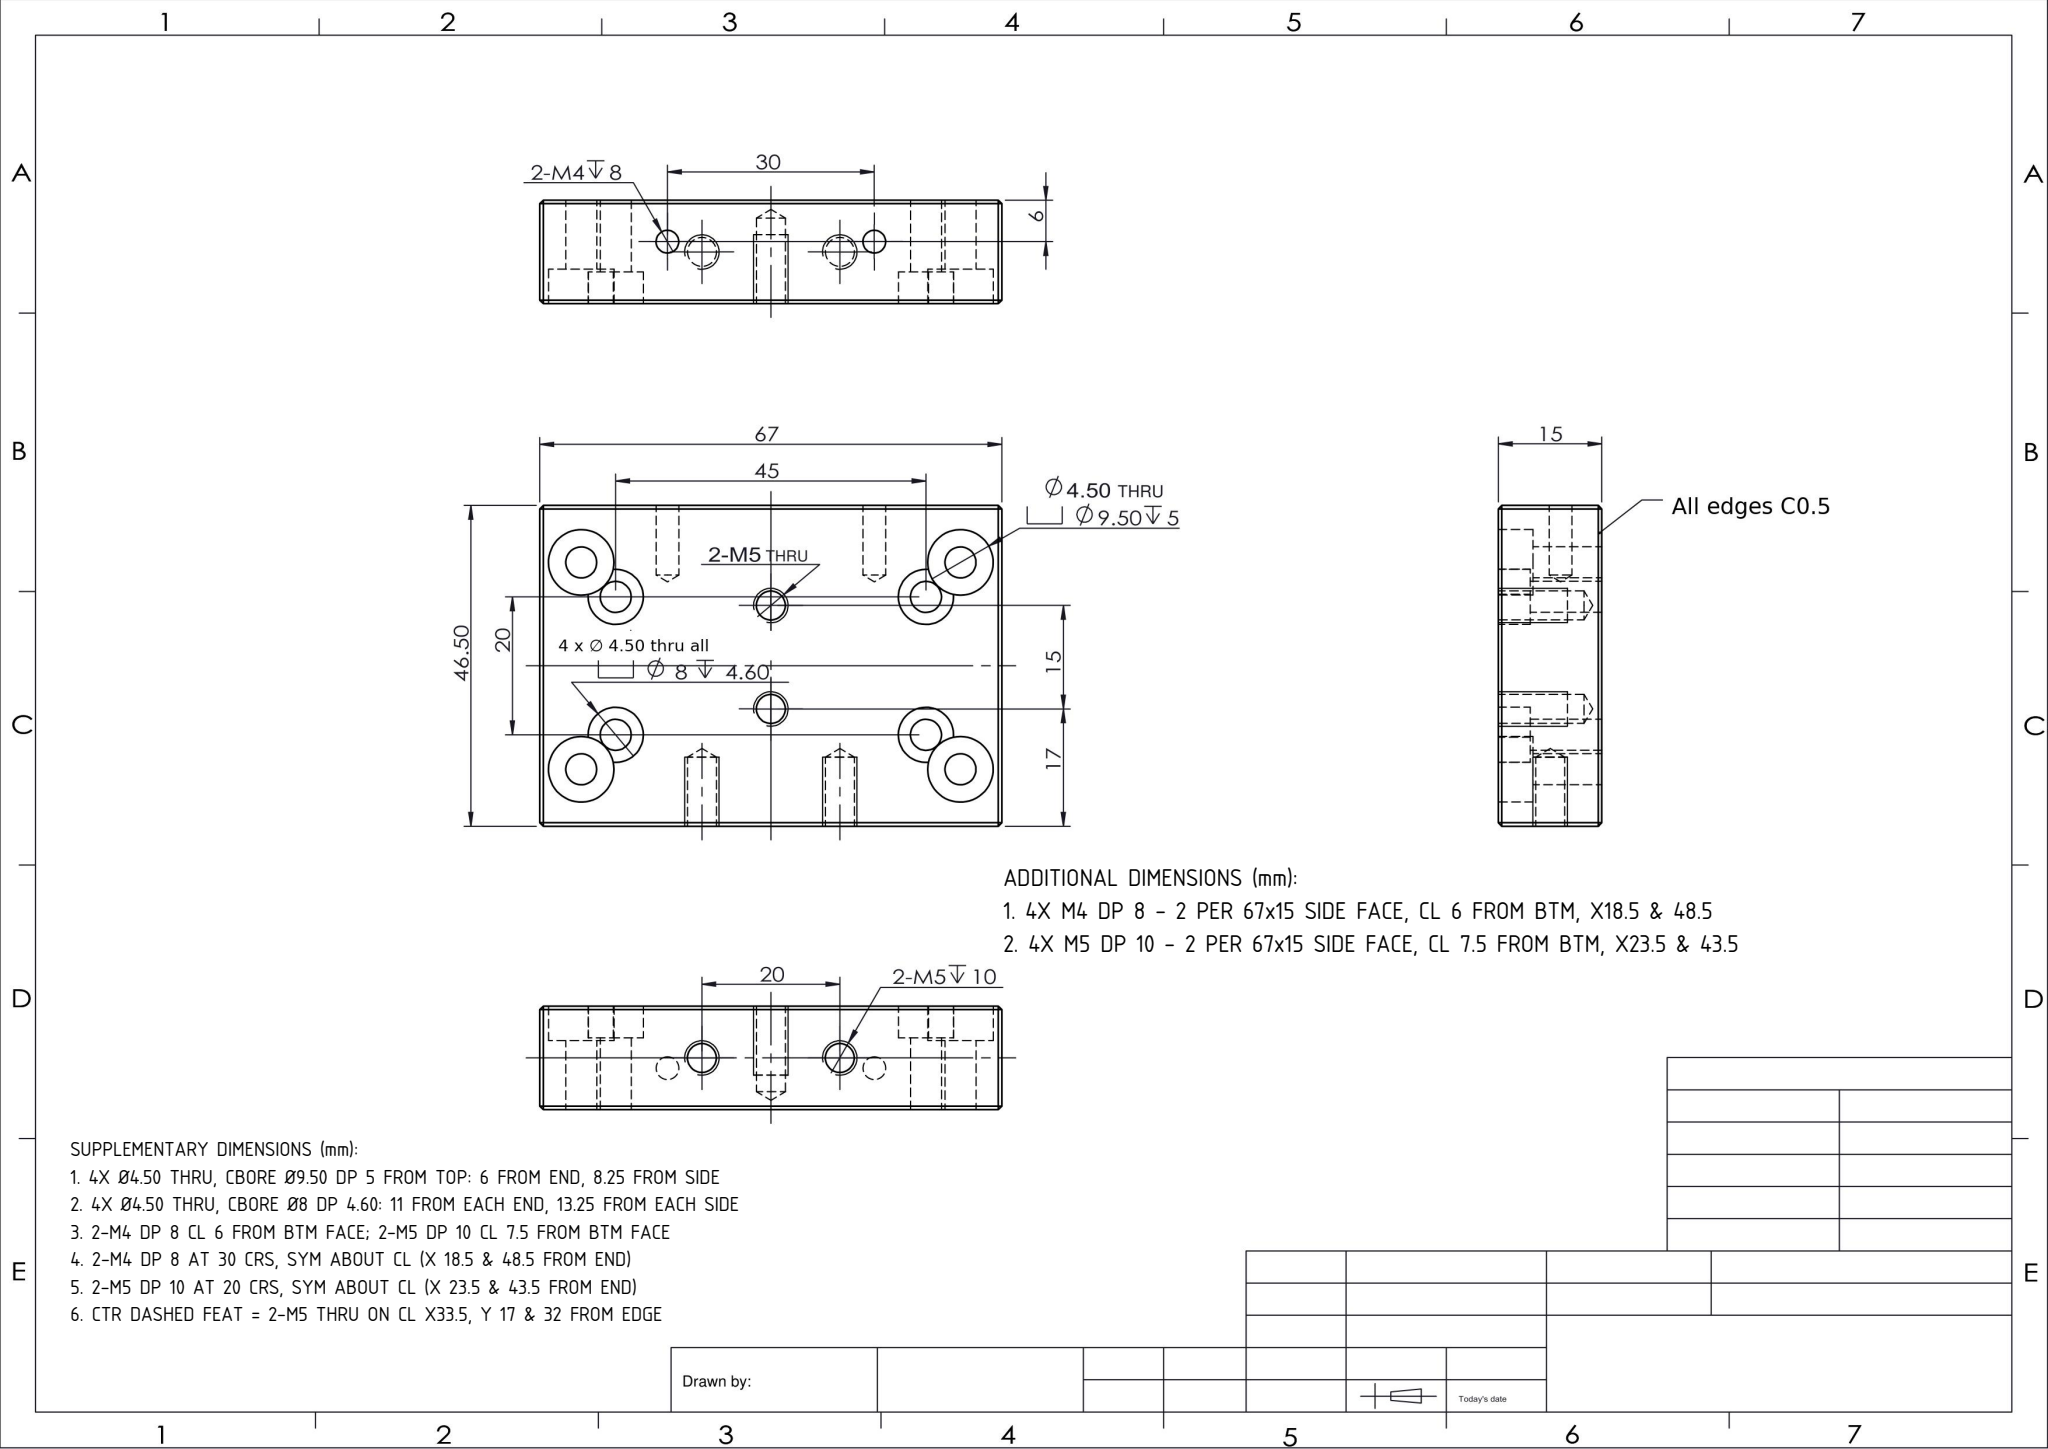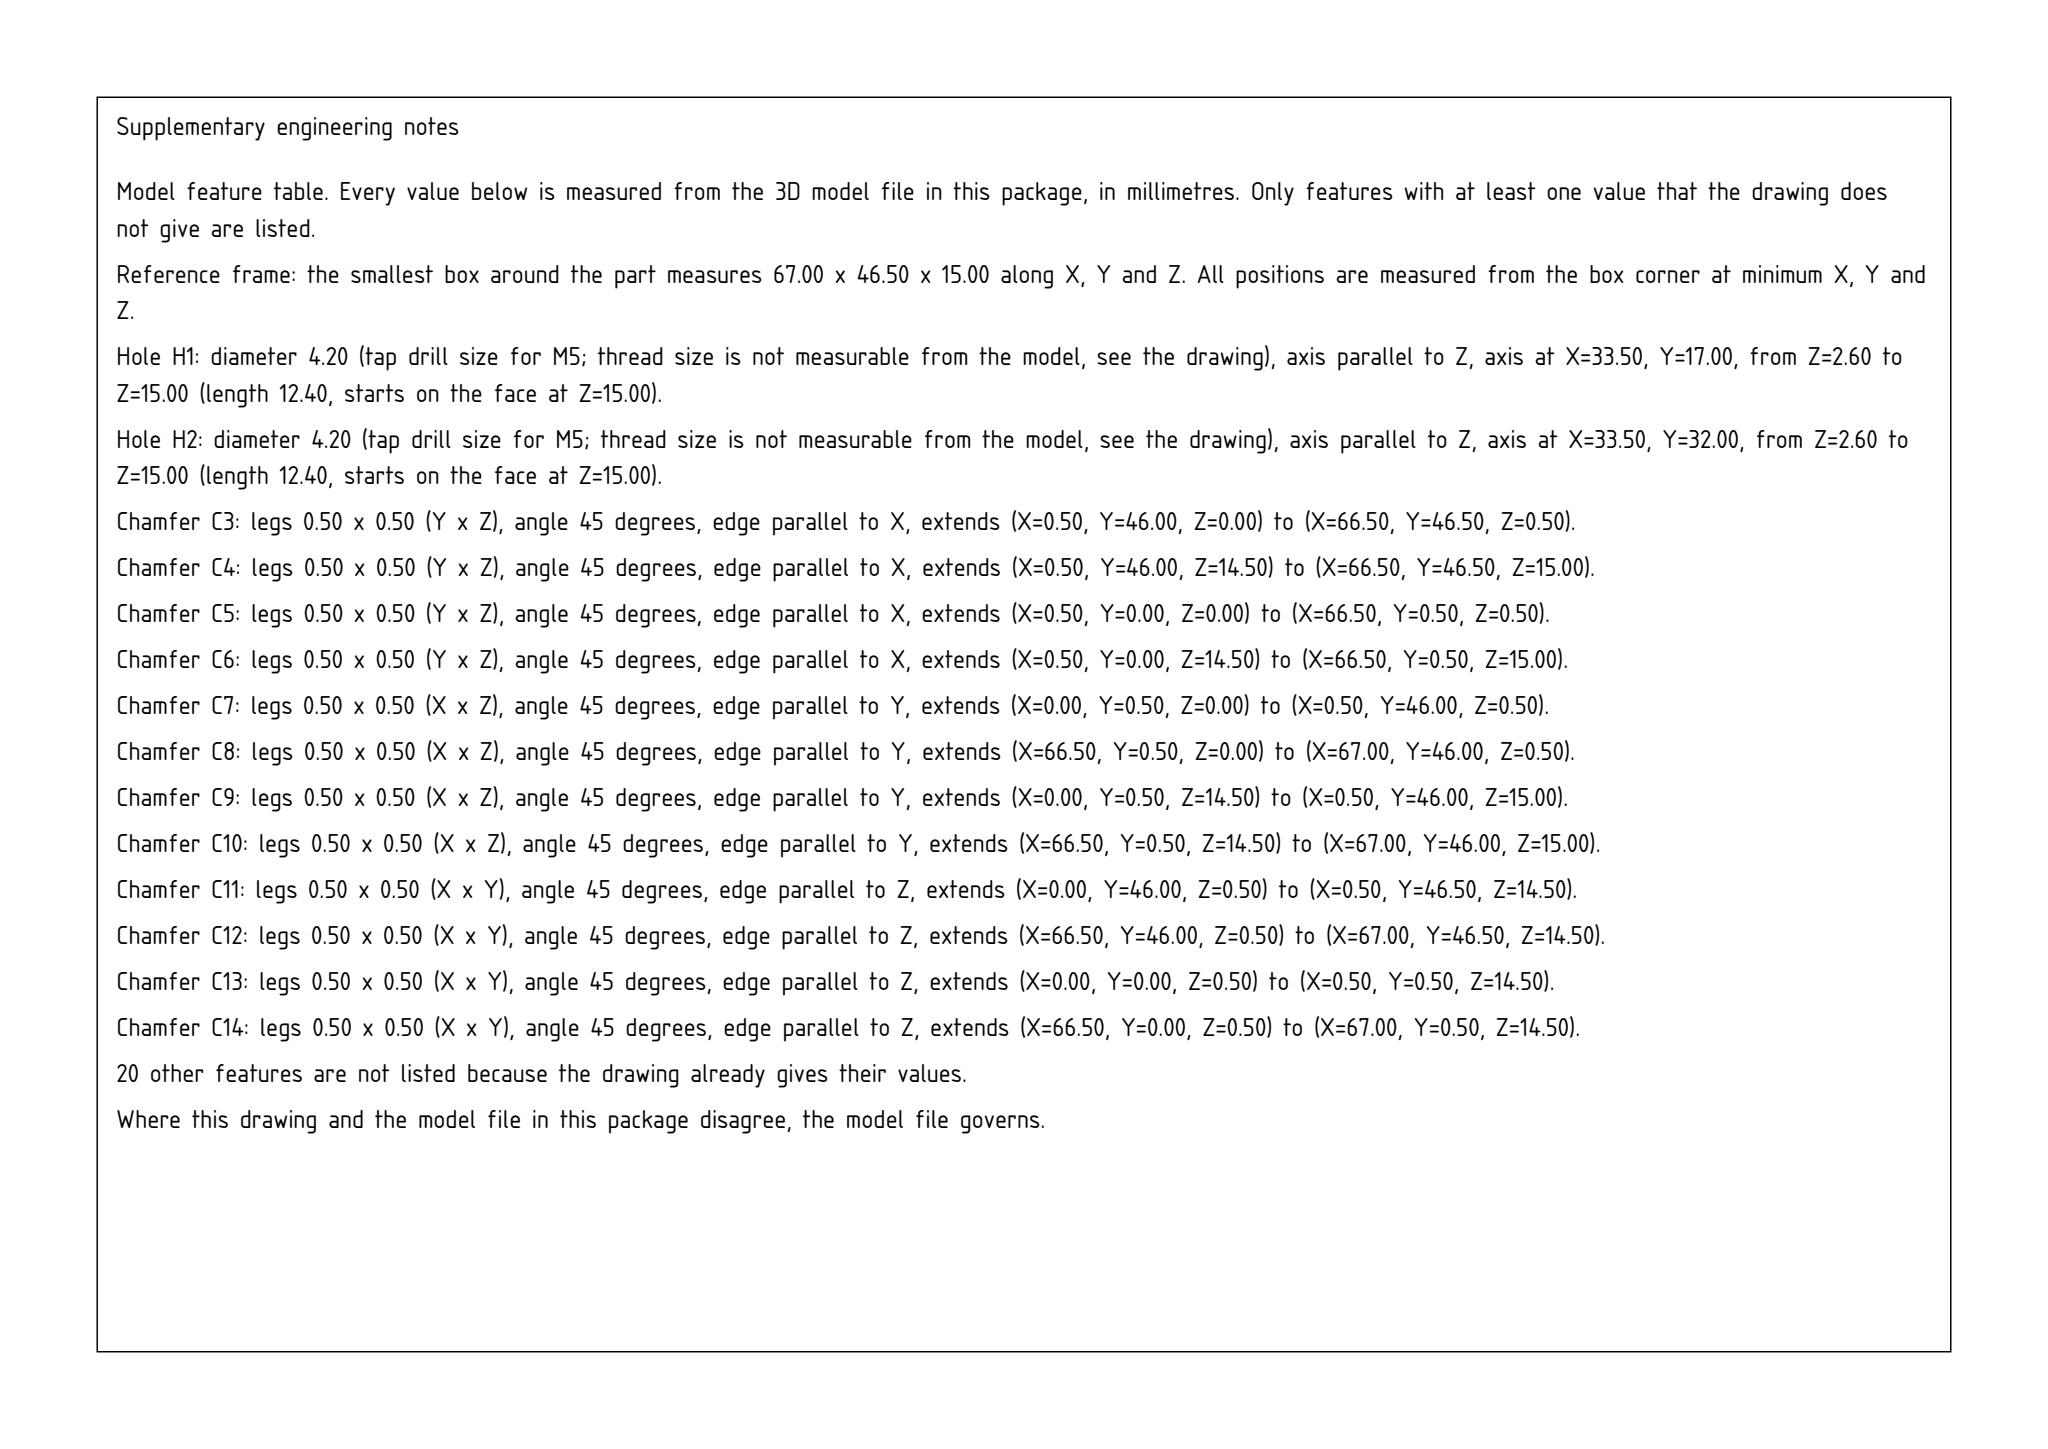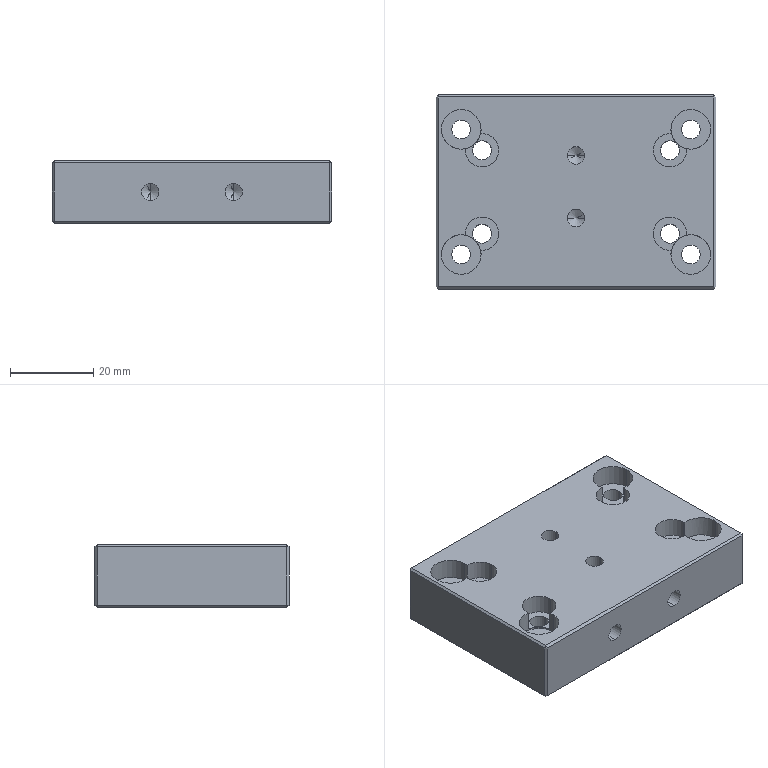Part | SolidWorks | mm | 1 solid | 94 faces | box 67 x 46.5 x 15 mm | volume 42314 mm3 | cylinder 48 | plane 34 | cone 12 | commonest cylinder face diameters 4.5 x16 8 x12 4.2 x8 9.5 x8 3.3 x4
build123d program:
from build123d import *

# Parameters (mm, degrees)
SKETCH1_W                                            = 67
SKETCH1_H                                            = 46.5
BOSS_EXTRUDE1_DEPTH                                  = 7.5
SKETCH2_R                                            = 2.25
CUT_EXTRUDE1_DEPTH                                   = 44.449
SKETCH3_R                                            = 4.75
CUT_EXTRUDE2_DEPTH                                   = 5
CHAMFER1_SIZE                                        = 0.5
M5_TAPPED_HOLE1_D                                    = 4.2
M5_TAPPED_HOLE1_DEPTH                                = 12.4
M5_TAPPED_HOLE1_TIP                                  = 1.262
M5_TAPPED_HOLE2_D                                    = 4.2
M5_TAPPED_HOLE2_DEPTH                                = 10
M5_TAPPED_HOLE2_TIP                                  = 1.262
M4_TAPPED_HOLE1_D                                    = 3.3
M4_TAPPED_HOLE1_DEPTH                                = 10.1
M4_TAPPED_HOLE1_TIP                                  = 0.9914
HOLE_SIZE_ACCORDING_TO_HEXAGON_SOCKET_HE_D           = 4.5
HOLE_SIZE_ACCORDING_TO_HEXAGON_SOCKET_HE_CBORE_D     = 8
HOLE_SIZE_ACCORDING_TO_HEXAGON_SOCKET_HE_CBORE_DEPTH = 4.6


with BuildPart() as part:
    # Sketch1 → Boss-Extrude1 (new, symmetric)
    with BuildSketch(Plane.XY):
        Rectangle(SKETCH1_W, SKETCH1_H)
    extrude(amount=BOSS_EXTRUDE1_DEPTH, both=True)

    # Sketch2 → Cut-Extrude1 (cut, through all)
    with BuildSketch(Plane.XY.offset(7.5)):
        with Locations((-27.5, 15)):
            Circle(SKETCH2_R)
        with Locations(Location((27.5, 15, 0), (0, 0, 180))):
            Circle(SKETCH2_R)
        with Locations((27.5, -15)):
            Circle(SKETCH2_R)
        with Locations(Location((-27.5, -15, 0), (0, 0, 180))):
            Circle(SKETCH2_R)
    extrude(amount=-CUT_EXTRUDE1_DEPTH, mode=Mode.SUBTRACT)

    # Sketch3 → Cut-Extrude2 (cut)
    with BuildSketch(Plane.XY.offset(7.5)):
        with Locations((-27.5, 15)):
            Circle(SKETCH3_R)
        with Locations((27.5, 15)):
            Circle(SKETCH3_R)
        with Locations((-27.5, -15)):
            Circle(SKETCH3_R)
        with Locations((27.5, -15)):
            Circle(SKETCH3_R)
    extrude(amount=-CUT_EXTRUDE2_DEPTH, mode=Mode.SUBTRACT)

    # Chamfer1
    chamfer1_edges = [part.edges().sort_by_distance(p)[0] for p in [
        (-33.5, 0, 7.5),
        (0, -23.25, 7.5),
        (33.5, 0, 7.5),
        (0, -23.25, -7.5),
        (-33.5, 0, -7.5),
        (0, 23.25, -7.5),
        (33.5, 0, -7.5),
        (0, 23.25, 7.5),
        (33.5, -23.25, 0),
        (-33.5, -23.25, 0),
        (-33.5, 23.25, 0),
        (33.5, 23.25, 0),
    ]]
    chamfer(chamfer1_edges, length=CHAMFER1_SIZE)

    # M5 Tapped Hole1
    with Locations(Plane.XY.offset(7.5)):
        with Locations((0, -6.25), (0, 8.75)):
            Hole(M5_TAPPED_HOLE1_D / 2, depth=M5_TAPPED_HOLE1_DEPTH)
            with Locations((0, 0, -(M5_TAPPED_HOLE1_DEPTH + M5_TAPPED_HOLE1_TIP / 2))):  # 118° drill point
                Cone(0, M5_TAPPED_HOLE1_D / 2, M5_TAPPED_HOLE1_TIP, mode=Mode.SUBTRACT)

    # M5 Tapped Hole2
    with Locations(Plane(origin=(0, -23.25, 0), x_dir=(-1, 0, 0), z_dir=(0, -1, 0))):
        with Locations((10, 0), (-10, 0)):
            Hole(M5_TAPPED_HOLE2_D / 2, depth=M5_TAPPED_HOLE2_DEPTH)
            with Locations((0, 0, -(M5_TAPPED_HOLE2_DEPTH + M5_TAPPED_HOLE2_TIP / 2))):  # 118° drill point
                Cone(0, M5_TAPPED_HOLE2_D / 2, M5_TAPPED_HOLE2_TIP, mode=Mode.SUBTRACT)

    # M4 Tapped Hole1
    with Locations(Plane(origin=(0, 23.25, 0), x_dir=(1, 0, 0), z_dir=(0, 1, 0))):
        with Locations((-15, 1.5), (15, 1.5)):
            Hole(M4_TAPPED_HOLE1_D / 2, depth=M4_TAPPED_HOLE1_DEPTH)
            with Locations((0, 0, -(M4_TAPPED_HOLE1_DEPTH + M4_TAPPED_HOLE1_TIP / 2))):  # 118° drill point
                Cone(0, M4_TAPPED_HOLE1_D / 2, M4_TAPPED_HOLE1_TIP, mode=Mode.SUBTRACT)

    # Hole Size according to Hexagon Socket He (through all)
    with Locations(Plane.XY.offset(7.5)):
        with Locations((-22.5, 10), (22.5, 10), (-22.5, -10), (22.5, -10)):
            CounterBoreHole(HOLE_SIZE_ACCORDING_TO_HEXAGON_SOCKET_HE_D / 2, HOLE_SIZE_ACCORDING_TO_HEXAGON_SOCKET_HE_CBORE_D / 2, HOLE_SIZE_ACCORDING_TO_HEXAGON_SOCKET_HE_CBORE_DEPTH)


solid = part.part